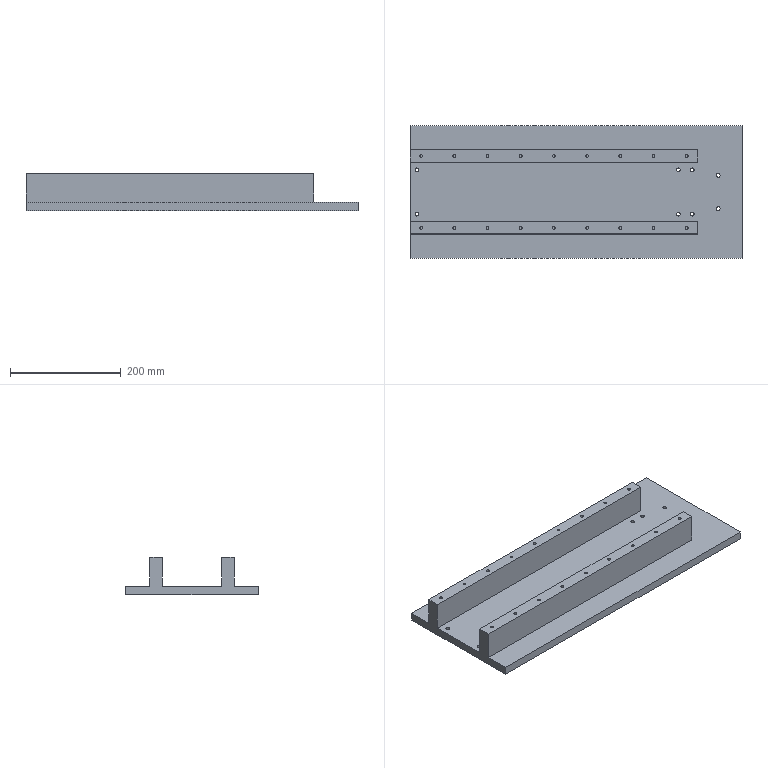Component | NX | GUIDE_RAIL_BASE_2 | 1 solid | 58 faces | volume 3339394 mm3 | plane 32 | cylinder 26 | commonest cylinder face diameters 5 x18 6.8 x8